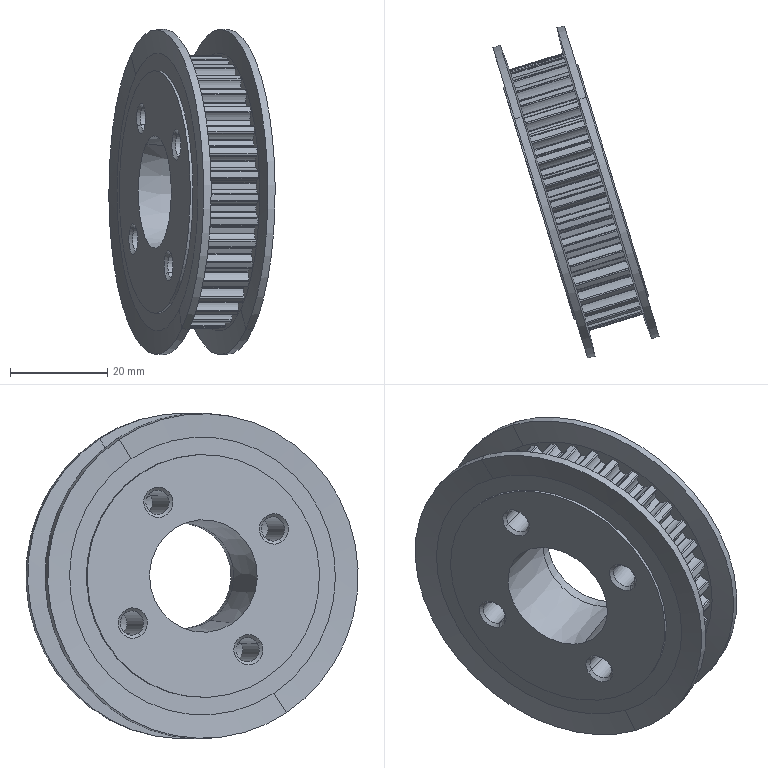Component | SolidWorks | v1ZHXTPTLA36P5M100_E_20SB1-1_v1ZHXTPTLA36P5M100_E_20_bodySB1-1 | 1 solid | 371 faces | box 34.22 x 68.39 x 67 mm | volume 33113 mm3 | cylinder 335 | cone 30 | plane 6 | commonest cylinder face diameters 0.5 x88 0.4 x82 6.64 x78 52.53 x37 56.15 x36 5.02 x8 50 x4 21.7 x2